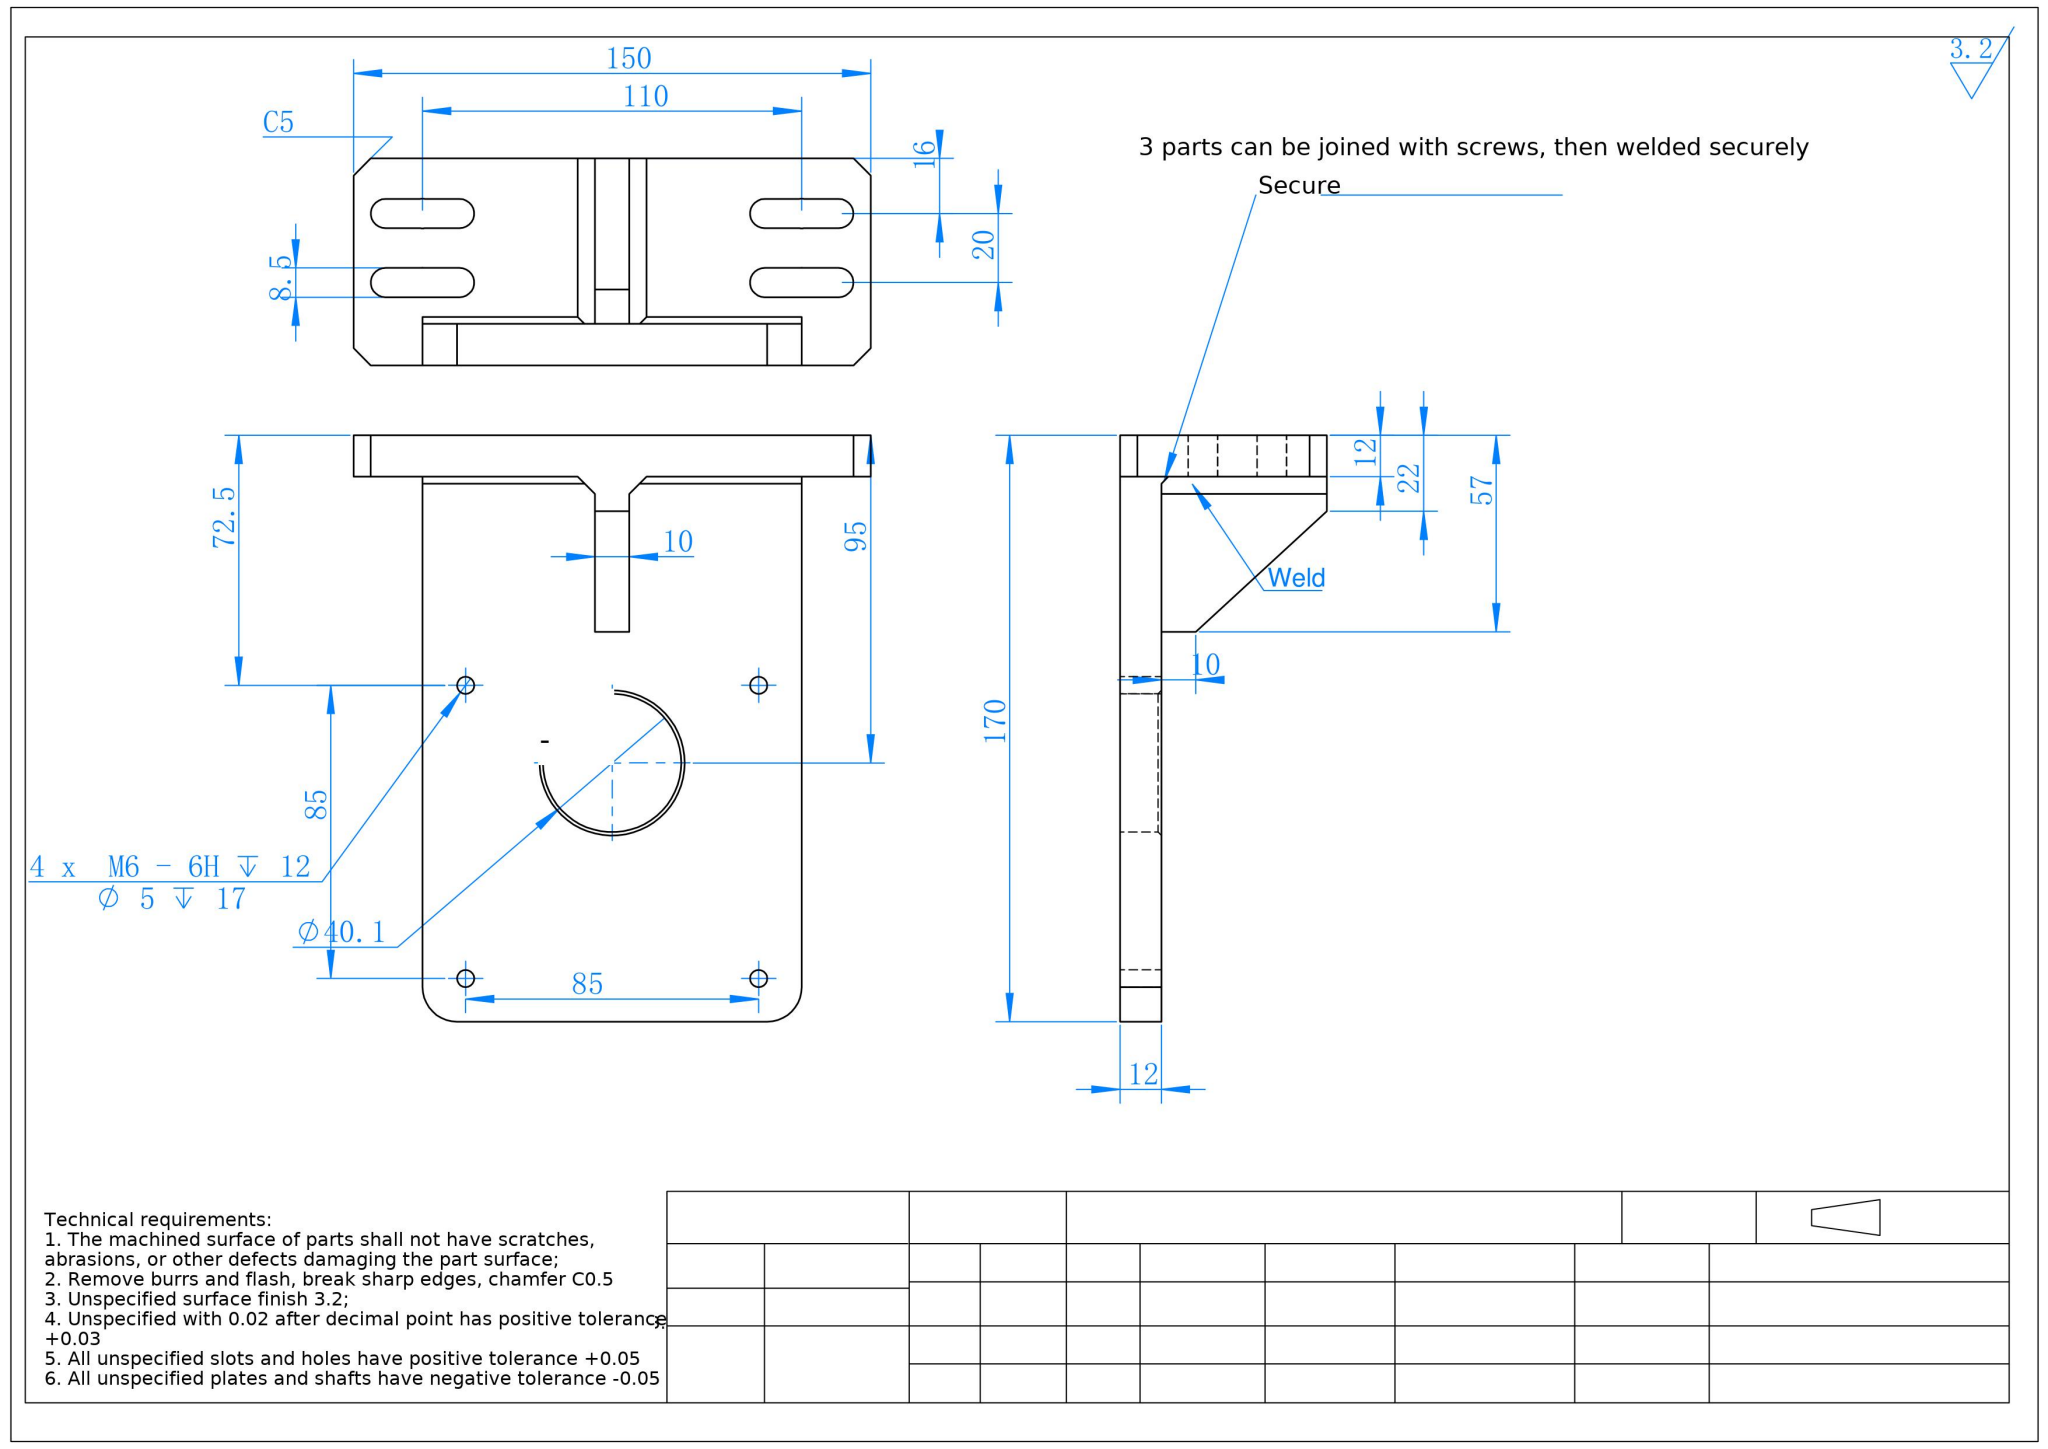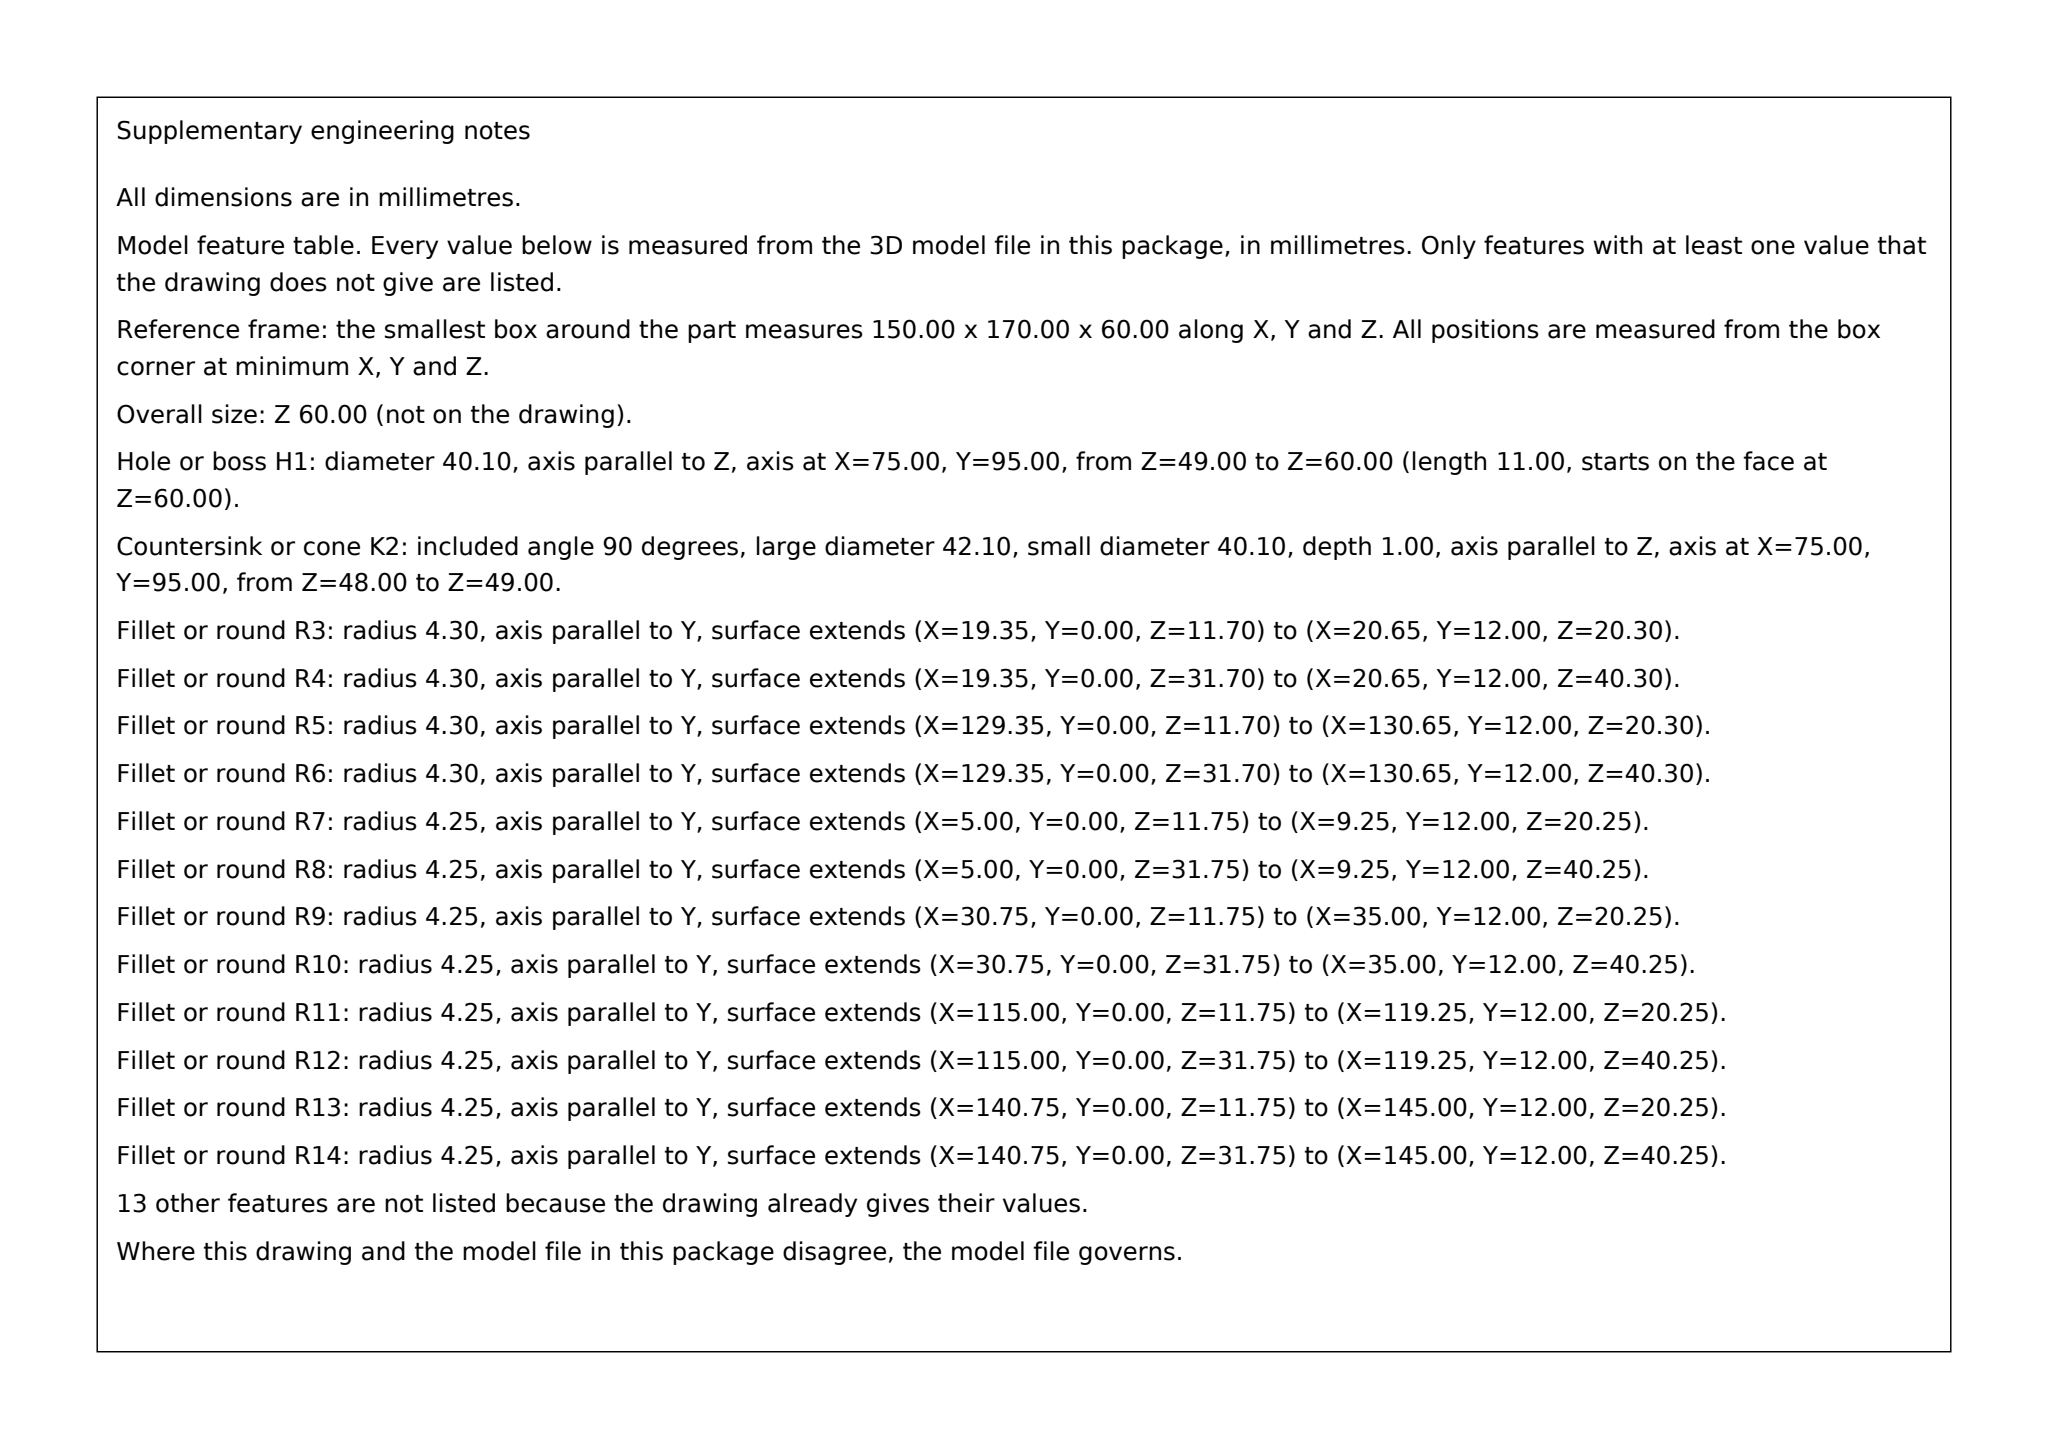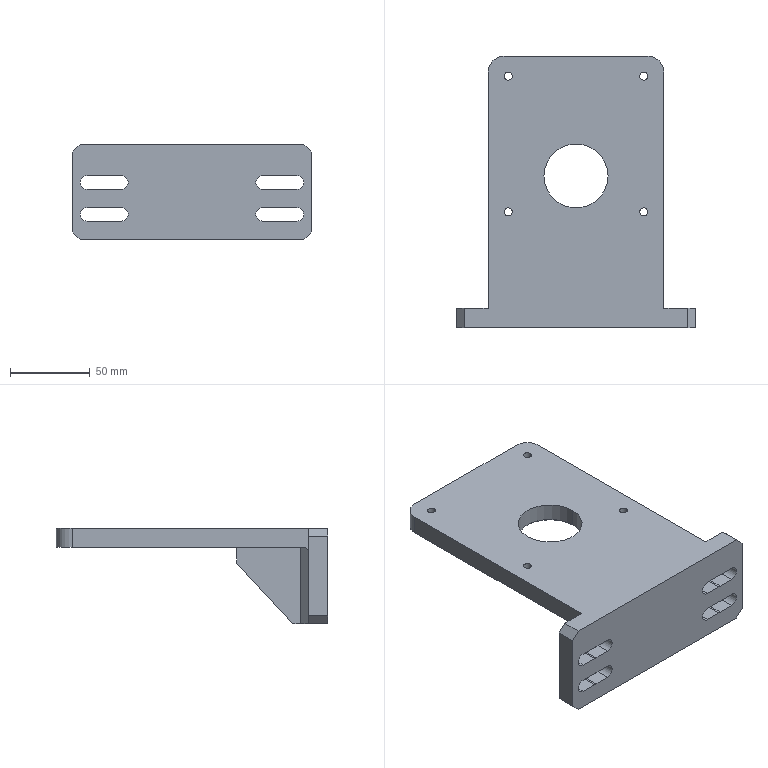Part | SolidWorks | mm | 1 solid | 73 faces | box 150 x 170 x 60 mm | volume 304116 mm3 | plane 39 | cylinder 32 | cone 2 | commonest cylinder face diameters 8.6 x12 5 x8 8.5 x8 40.1 x2 20 x2